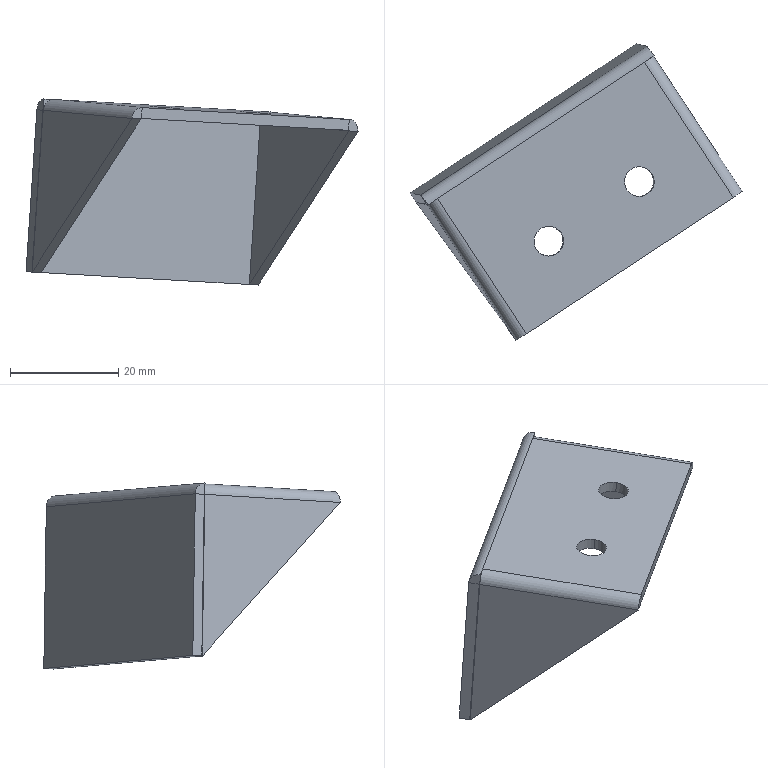Component | SolidWorks | LinearGuideRodSheetMetal-1 | 1 solid | 34 faces | box 61.25 x 54.67 x 34.32 mm | volume 7801 mm3 | plane 24 | cylinder 10 | commonest cylinder face diameters 5.5 x4 0.2 x3 4.2 x3 | material AISI 304
STEP:
#1=COLOUR_RGB('',0.7922,0.8196,0.9333);
#2=FILL_AREA_STYLE_COLOUR('',#1);
#3=FILL_AREA_STYLE('',(#2));
#4=SURFACE_STYLE_FILL_AREA(#3);
#5=SURFACE_SIDE_STYLE('',(#4));
#6=SURFACE_STYLE_USAGE(.BOTH.,#5);
#7=PRESENTATION_STYLE_ASSIGNMENT((#6));
#8=CARTESIAN_POINT('',(-6.363,-0.1525,32.19));
#9=VERTEX_POINT('',#8);
#10=CARTESIAN_POINT('',(-6.182,-0.03352,32.18));
#11=VERTEX_POINT('',#10);
#12=CARTESIAN_POINT('',(-6.272,-0.09302,32.185));
#13=DIRECTION('',(-0.0675,0.01553,-0.9976));
#14=DIRECTION('',(-0.8341,-0.5496,0.04788));
#15=AXIS2_PLACEMENT_3D('',#12,#13,#14);
#16=CIRCLE('',#15,0.1083);
#17=EDGE_CURVE('',#9,#11,#16,.T.);
#18=ORIENTED_EDGE('',*,*,#17,.T.);
#19=CARTESIAN_POINT('',(-6.177,-0.03474,32.258));
#20=VERTEX_POINT('',#19);
#21=CARTESIAN_POINT('',(-6.182,-0.03352,32.18));
#22=DIRECTION('',(0.0675,-0.01553,0.9976));
#23=VECTOR('',#22,39.37);
#24=LINE('',#21,#23);
#25=EDGE_CURVE('',#11,#20,#24,.T.);
#26=ORIENTED_EDGE('',*,*,#25,.T.);
#27=CARTESIAN_POINT('',(-6.357,-0.1537,32.269));
#28=VERTEX_POINT('',#27);
#29=CARTESIAN_POINT('',(-6.267,-0.09424,32.264));
#30=DIRECTION('',(-0.0675,0.01553,-0.9976));
#31=DIRECTION('',(-0.8341,-0.5496,0.04788));
#32=AXIS2_PLACEMENT_3D('',#29,#30,#31);
#33=CIRCLE('',#32,0.1083);
#34=EDGE_CURVE('',#28,#20,#33,.T.);
#35=ORIENTED_EDGE('',*,*,#34,.F.);
#36=CARTESIAN_POINT('',(-6.363,-0.1525,32.19));
#37=DIRECTION('',(0.0675,-0.01553,0.9976));
#38=VECTOR('',#37,39.37);
#39=LINE('',#36,#38);
#40=EDGE_CURVE('',#9,#28,#39,.T.);
#41=ORIENTED_EDGE('',*,*,#40,.F.);
#42=EDGE_LOOP('',(#18,#26,#35,#41));
#43=FACE_OUTER_BOUND('',#42,.T.);
#44=CARTESIAN_POINT('',(-6.272,-0.09302,32.185));
#45=DIRECTION('',(0.0675,-0.01553,0.9976));
#46=DIRECTION('',(-0.8341,-0.5496,0.04788));
#47=AXIS2_PLACEMENT_3D('',#44,#45,#46);
#48=CYLINDRICAL_SURFACE('',#47,0.1083);
#49=ADVANCED_FACE('',(#43),#48,.F.);
#50=CARTESIAN_POINT('',(-5.706,0.2802,32.152));
#51=VERTEX_POINT('',#50);
#52=CARTESIAN_POINT('',(-5.525,0.3992,32.142));
#53=VERTEX_POINT('',#52);
#54=CARTESIAN_POINT('',(-5.616,0.3397,32.147));
#55=DIRECTION('',(-0.0675,0.01553,-0.9976));
#56=DIRECTION('',(-0.8341,-0.5496,0.04788));
#57=AXIS2_PLACEMENT_3D('',#54,#55,#56);
#58=CIRCLE('',#57,0.1083);
#59=EDGE_CURVE('',#51,#53,#58,.T.);
#60=ORIENTED_EDGE('',*,*,#59,.T.);
#61=CARTESIAN_POINT('',(-5.52,0.398,32.221));
#62=VERTEX_POINT('',#61);
#63=CARTESIAN_POINT('',(-5.525,0.3992,32.142));
#64=DIRECTION('',(0.0675,-0.01553,0.9976));
#65=VECTOR('',#64,39.37);
#66=LINE('',#63,#65);
#67=EDGE_CURVE('',#53,#62,#66,.T.);
#68=ORIENTED_EDGE('',*,*,#67,.T.);
#69=CARTESIAN_POINT('',(-5.701,0.279,32.231));
#70=VERTEX_POINT('',#69);
#71=CARTESIAN_POINT('',(-5.61,0.3385,32.226));
#72=DIRECTION('',(-0.0675,0.01553,-0.9976));
#73=DIRECTION('',(-0.8341,-0.5496,0.04788));
#74=AXIS2_PLACEMENT_3D('',#71,#72,#73);
#75=CIRCLE('',#74,0.1083);
#76=EDGE_CURVE('',#70,#62,#75,.T.);
#77=ORIENTED_EDGE('',*,*,#76,.F.);
#78=CARTESIAN_POINT('',(-5.706,0.2802,32.152));
#79=DIRECTION('',(0.0675,-0.01553,0.9976));
#80=VECTOR('',#79,39.37);
#81=LINE('',#78,#80);
#82=EDGE_CURVE('',#51,#70,#81,.T.);
#83=ORIENTED_EDGE('',*,*,#82,.F.);
#84=EDGE_LOOP('',(#60,#68,#77,#83));
#85=FACE_OUTER_BOUND('',#84,.T.);
#86=CARTESIAN_POINT('',(-5.616,0.3397,32.147));
#87=DIRECTION('',(0.0675,-0.01553,0.9976));
#88=DIRECTION('',(-0.8341,-0.5496,0.04788));
#89=AXIS2_PLACEMENT_3D('',#86,#87,#88);
#90=CYLINDRICAL_SURFACE('',#89,0.1083);
#91=ADVANCED_FACE('',(#85),#90,.F.);
#92=CARTESIAN_POINT('',(-5.572,1.206,32.237));
#93=VERTEX_POINT('',#92);
#94=CARTESIAN_POINT('',(-5.504,1.252,32.233));
#95=VERTEX_POINT('',#94);
#96=CARTESIAN_POINT('',(-7.145,0.1699,32.327));
#97=DIRECTION('',(0.8341,0.5496,-0.04788));
#98=VECTOR('',#97,39.37);
#99=LINE('',#96,#98);
#100=EDGE_CURVE('',#93,#95,#99,.T.);
#101=ORIENTED_EDGE('',*,*,#100,.F.);
#102=CARTESIAN_POINT('',(-5.509,1.253,32.154));
#103=VERTEX_POINT('',#102);
#104=CARTESIAN_POINT('',(-5.578,1.208,32.154));
#105=DIRECTION('',(-0.5475,0.8353,0.05005));
#106=DIRECTION('',(0.8341,0.5496,-0.04788));
#107=AXIS2_PLACEMENT_3D('',#104,#105,#106);
#108=CIRCLE('',#107,0.08268);
#109=EDGE_CURVE('',#93,#103,#108,.T.);
#110=ORIENTED_EDGE('',*,*,#109,.T.);
#111=CARTESIAN_POINT('',(-5.509,1.253,32.154));
#112=VERTEX_POINT('',#111);
#113=CARTESIAN_POINT('',(-5.578,1.207,32.158));
#114=DIRECTION('',(0.8341,0.5496,-0.04788));
#115=VECTOR('',#114,39.37);
#116=LINE('',#113,#115);
#117=EDGE_CURVE('',#103,#112,#116,.T.);
#118=ORIENTED_EDGE('',*,*,#117,.T.);
#119=CARTESIAN_POINT('',(-5.509,1.253,32.154));
#120=DIRECTION('',(-0.0675,0.01553,-0.9976));
#121=VECTOR('',#120,39.37);
#122=LINE('',#119,#121);
#123=EDGE_CURVE('',#95,#112,#122,.T.);
#124=ORIENTED_EDGE('',*,*,#123,.F.);
#125=EDGE_LOOP('',(#101,#110,#118,#124));
#126=FACE_OUTER_BOUND('',#125,.T.);
#127=CARTESIAN_POINT('',(-5.578,1.207,32.158));
#128=DIRECTION('',(0.5475,-0.8353,-0.05005));
#129=DIRECTION('',(0.8341,0.5496,-0.04788));
#130=AXIS2_PLACEMENT_3D('',#127,#128,#129);
#131=PLANE('',#130);
#132=ADVANCED_FACE('',(#126),#131,.T.);
#133=CARTESIAN_POINT('',(-7.151,0.1711,32.249));
#134=VERTEX_POINT('',#133);
#135=CARTESIAN_POINT('',(-7.151,0.1711,32.249));
#136=VERTEX_POINT('',#135);
#137=CARTESIAN_POINT('',(-5.509,1.253,32.154));
#138=DIRECTION('',(0.8341,0.5496,-0.04788));
#139=VECTOR('',#138,39.37);
#140=LINE('',#137,#139);
#141=EDGE_CURVE('',#134,#136,#140,.T.);
#142=ORIENTED_EDGE('',*,*,#141,.T.);
#143=CARTESIAN_POINT('',(-7.076,0.2153,32.323));
#144=VERTEX_POINT('',#143);
#145=CARTESIAN_POINT('',(-7.082,0.2166,32.241));
#146=DIRECTION('',(-0.5475,0.8353,0.05005));
#147=DIRECTION('',(-0.8341,-0.5496,0.04788));
#148=AXIS2_PLACEMENT_3D('',#145,#146,#147);
#149=CIRCLE('',#148,0.08268);
#150=EDGE_CURVE('',#136,#144,#149,.T.);
#151=ORIENTED_EDGE('',*,*,#150,.T.);
#152=CARTESIAN_POINT('',(-7.145,0.1699,32.327));
#153=VERTEX_POINT('',#152);
#154=CARTESIAN_POINT('',(-7.145,0.1699,32.327));
#155=DIRECTION('',(0.8341,0.5496,-0.04788));
#156=VECTOR('',#155,39.37);
#157=LINE('',#154,#156);
#158=EDGE_CURVE('',#153,#144,#157,.T.);
#159=ORIENTED_EDGE('',*,*,#158,.F.);
#160=CARTESIAN_POINT('',(-7.151,0.1711,32.249));
#161=DIRECTION('',(-0.0675,0.01553,-0.9976));
#162=VECTOR('',#161,39.37);
#163=LINE('',#160,#162);
#164=EDGE_CURVE('',#153,#134,#163,.T.);
#165=ORIENTED_EDGE('',*,*,#164,.T.);
#166=EDGE_LOOP('',(#142,#151,#159,#165));
#167=FACE_OUTER_BOUND('',#166,.T.);
#168=CARTESIAN_POINT('',(-7.151,0.1711,32.249));
#169=DIRECTION('',(0.5475,-0.8353,-0.05005));
#170=DIRECTION('',(0.8341,0.5496,-0.04788));
#171=AXIS2_PLACEMENT_3D('',#168,#169,#170);
#172=PLANE('',#171);
#173=ADVANCED_FACE('',(#167),#172,.T.);
#174=ORIENTED_EDGE('',*,*,#59,.F.);
#175=CARTESIAN_POINT('',(-5.616,0.3397,32.147));
#176=DIRECTION('',(-0.0675,0.01553,-0.9976));
#177=DIRECTION('',(-0.8341,-0.5496,0.04788));
#178=AXIS2_PLACEMENT_3D('',#175,#176,#177);
#179=CIRCLE('',#178,0.1083);
#180=EDGE_CURVE('',#53,#51,#179,.T.);
#181=ORIENTED_EDGE('',*,*,#180,.F.);
#182=EDGE_LOOP('',(#174,#181));
#183=FACE_BOUND('',#182,.T.);
#184=ORIENTED_EDGE('',*,*,#17,.F.);
#185=CARTESIAN_POINT('',(-6.272,-0.09302,32.185));
#186=DIRECTION('',(-0.0675,0.01553,-0.9976));
#187=DIRECTION('',(-0.8341,-0.5496,0.04788));
#188=AXIS2_PLACEMENT_3D('',#185,#186,#187);
#189=CIRCLE('',#188,0.1083);
#190=EDGE_CURVE('',#11,#9,#189,.T.);
#191=ORIENTED_EDGE('',*,*,#190,.F.);
#192=EDGE_LOOP('',(#184,#191));
#193=FACE_BOUND('',#192,.T.);
#194=CARTESIAN_POINT('',(-4.933,0.2242,32.099));
#195=VERTEX_POINT('',#194);
#196=CARTESIAN_POINT('',(-5.578,1.207,32.158));
#197=VERTEX_POINT('',#196);
#198=CARTESIAN_POINT('',(-4.933,0.2242,32.099));
#199=DIRECTION('',(-0.5475,0.8353,0.05005));
#200=VECTOR('',#199,39.37);
#201=LINE('',#198,#200);
#202=EDGE_CURVE('',#195,#197,#201,.T.);
#203=ORIENTED_EDGE('',*,*,#202,.F.);
#204=CARTESIAN_POINT('',(-6.437,-0.7668,32.186));
#205=VERTEX_POINT('',#204);
#206=CARTESIAN_POINT('',(-6.506,-0.8122,32.19));
#207=DIRECTION('',(0.8341,0.5496,-0.04788));
#208=VECTOR('',#207,39.37);
#209=LINE('',#206,#208);
#210=EDGE_CURVE('',#205,#195,#209,.T.);
#211=ORIENTED_EDGE('',*,*,#210,.F.);
#212=CARTESIAN_POINT('',(-7.082,0.2165,32.245));
#213=VERTEX_POINT('',#212);
#214=CARTESIAN_POINT('',(-7.082,0.2165,32.245));
#215=DIRECTION('',(0.5475,-0.8353,-0.05005));
#216=VECTOR('',#215,39.37);
#217=LINE('',#214,#216);
#218=EDGE_CURVE('',#213,#205,#217,.T.);
#219=ORIENTED_EDGE('',*,*,#218,.F.);
#220=CARTESIAN_POINT('',(-5.509,1.253,32.154));
#221=DIRECTION('',(0.8341,0.5496,-0.04788));
#222=VECTOR('',#221,39.37);
#223=LINE('',#220,#222);
#224=EDGE_CURVE('',#213,#197,#223,.T.);
#225=ORIENTED_EDGE('',*,*,#224,.T.);
#226=EDGE_LOOP('',(#203,#211,#219,#225));
#227=FACE_OUTER_BOUND('',#226,.T.);
#228=CARTESIAN_POINT('',(-7.153,0.1744,32.249));
#229=DIRECTION('',(0.0675,-0.01553,0.9976));
#230=DIRECTION('',(-0.8341,-0.5496,0.04788));
#231=AXIS2_PLACEMENT_3D('',#228,#229,#230);
#232=PLANE('',#231);
#233=ADVANCED_FACE('',(#183,#193,#227),#232,.F.);
#234=ORIENTED_EDGE('',*,*,#76,.T.);
#235=CARTESIAN_POINT('',(-5.61,0.3385,32.226));
#236=DIRECTION('',(-0.0675,0.01553,-0.9976));
#237=DIRECTION('',(-0.8341,-0.5496,0.04788));
#238=AXIS2_PLACEMENT_3D('',#235,#236,#237);
#239=CIRCLE('',#238,0.1083);
#240=EDGE_CURVE('',#62,#70,#239,.T.);
#241=ORIENTED_EDGE('',*,*,#240,.T.);
#242=EDGE_LOOP('',(#234,#241));
#243=FACE_BOUND('',#242,.T.);
#244=ORIENTED_EDGE('',*,*,#34,.T.);
#245=CARTESIAN_POINT('',(-6.267,-0.09424,32.264));
#246=DIRECTION('',(-0.0675,0.01553,-0.9976));
#247=DIRECTION('',(-0.8341,-0.5496,0.04788));
#248=AXIS2_PLACEMENT_3D('',#245,#246,#247);
#249=CIRCLE('',#248,0.1083);
#250=EDGE_CURVE('',#20,#28,#249,.T.);
#251=ORIENTED_EDGE('',*,*,#250,.T.);
#252=EDGE_LOOP('',(#244,#251));
#253=FACE_BOUND('',#252,.T.);
#254=CARTESIAN_POINT('',(-6.432,-0.768,32.264));
#255=VERTEX_POINT('',#254);
#256=CARTESIAN_POINT('',(-4.928,0.223,32.178));
#257=VERTEX_POINT('',#256);
#258=CARTESIAN_POINT('',(-6.501,-0.8134,32.268));
#259=DIRECTION('',(0.8341,0.5496,-0.04788));
#260=VECTOR('',#259,39.37);
#261=LINE('',#258,#260);
#262=EDGE_CURVE('',#255,#257,#261,.T.);
#263=ORIENTED_EDGE('',*,*,#262,.T.);
#264=CARTESIAN_POINT('',(-4.928,0.223,32.178));
#265=DIRECTION('',(-0.5475,0.8353,0.05005));
#266=VECTOR('',#265,39.37);
#267=LINE('',#264,#266);
#268=EDGE_CURVE('',#257,#93,#267,.T.);
#269=ORIENTED_EDGE('',*,*,#268,.T.);
#270=CARTESIAN_POINT('',(-7.145,0.1699,32.327));
#271=DIRECTION('',(0.8341,0.5496,-0.04788));
#272=VECTOR('',#271,39.37);
#273=LINE('',#270,#272);
#274=EDGE_CURVE('',#144,#93,#273,.T.);
#275=ORIENTED_EDGE('',*,*,#274,.F.);
#276=CARTESIAN_POINT('',(-7.076,0.2153,32.323));
#277=DIRECTION('',(0.5475,-0.8353,-0.05005));
#278=VECTOR('',#277,39.37);
#279=LINE('',#276,#278);
#280=EDGE_CURVE('',#144,#255,#279,.T.);
#281=ORIENTED_EDGE('',*,*,#280,.T.);
#282=EDGE_LOOP('',(#263,#269,#275,#281));
#283=FACE_OUTER_BOUND('',#282,.T.);
#284=CARTESIAN_POINT('',(-7.148,0.1731,32.327));
#285=DIRECTION('',(0.0675,-0.01553,0.9976));
#286=DIRECTION('',(-0.8341,-0.5496,0.04788));
#287=AXIS2_PLACEMENT_3D('',#284,#285,#286);
#288=PLANE('',#287);
#289=ADVANCED_FACE('',(#243,#253,#283),#288,.T.);
#290=ORIENTED_EDGE('',*,*,#210,.T.);
#291=CARTESIAN_POINT('',(-4.933,0.2242,32.099));
#292=DIRECTION('',(0.0675,-0.01553,0.9976));
#293=VECTOR('',#292,39.37);
#294=LINE('',#291,#293);
#295=EDGE_CURVE('',#195,#257,#294,.T.);
#296=ORIENTED_EDGE('',*,*,#295,.T.);
#297=ORIENTED_EDGE('',*,*,#262,.F.);
#298=CARTESIAN_POINT('',(-6.437,-0.7668,32.186));
#299=DIRECTION('',(0.0675,-0.01553,0.9976));
#300=VECTOR('',#299,39.37);
#301=LINE('',#298,#300);
#302=EDGE_CURVE('',#205,#255,#301,.T.);
#303=ORIENTED_EDGE('',*,*,#302,.F.);
#304=EDGE_LOOP('',(#290,#296,#297,#303));
#305=FACE_OUTER_BOUND('',#304,.T.);
#306=CARTESIAN_POINT('',(-6.506,-0.8122,32.19));
#307=DIRECTION('',(0.5475,-0.8353,-0.05005));
#308=DIRECTION('',(0.8341,0.5496,-0.04788));
#309=AXIS2_PLACEMENT_3D('',#306,#307,#308);
#310=PLANE('',#309);
#311=ADVANCED_FACE('',(#305),#310,.T.);
#312=ORIENTED_EDGE('',*,*,#164,.F.);
#313=CARTESIAN_POINT('',(-7.196,0.2402,32.249));
#314=VERTEX_POINT('',#313);
#315=CARTESIAN_POINT('',(-7.151,0.1711,32.245));
#316=DIRECTION('',(-0.8341,-0.5496,0.04788));
#317=DIRECTION('',(0.5475,-0.8353,-0.05005));
#318=AXIS2_PLACEMENT_3D('',#315,#316,#317);
#319=CIRCLE('',#318,0.08268);
#320=EDGE_CURVE('',#153,#314,#319,.T.);
#321=ORIENTED_EDGE('',*,*,#320,.T.);
#322=CARTESIAN_POINT('',(-7.153,0.1744,32.245));
#323=VERTEX_POINT('',#322);
#324=CARTESIAN_POINT('',(-7.153,0.1744,32.245));
#325=DIRECTION('',(0.5475,-0.8353,-0.05005));
#326=VECTOR('',#325,39.37);
#327=LINE('',#324,#326);
#328=EDGE_CURVE('',#314,#323,#327,.T.);
#329=ORIENTED_EDGE('',*,*,#328,.T.);
#330=CARTESIAN_POINT('',(-7.151,0.1711,32.245));
#331=DIRECTION('',(-0.8341,-0.5496,0.04788));
#332=DIRECTION('',(-0.5475,0.8353,0.05005));
#333=AXIS2_PLACEMENT_3D('',#330,#331,#332);
#334=CIRCLE('',#333,0.003937);
#335=EDGE_CURVE('',#134,#323,#334,.T.);
#336=ORIENTED_EDGE('',*,*,#335,.F.);
#337=EDGE_LOOP('',(#312,#321,#329,#336));
#338=FACE_OUTER_BOUND('',#337,.T.);
#339=CARTESIAN_POINT('',(-7.151,0.1711,32.245));
#340=DIRECTION('',(-0.8341,-0.5496,0.04788));
#341=DIRECTION('',(0.5475,-0.8353,-0.05005));
#342=AXIS2_PLACEMENT_3D('',#339,#340,#341);
#343=PLANE('',#342);
#344=ADVANCED_FACE('',(#338),#343,.T.);
#345=ORIENTED_EDGE('',*,*,#328,.F.);
#346=CARTESIAN_POINT('',(-7.276,0.2585,31.074));
#347=VERTEX_POINT('',#346);
#348=CARTESIAN_POINT('',(-7.196,0.2401,32.253));
#349=DIRECTION('',(0.0675,-0.01553,0.9976));
#350=VECTOR('',#349,39.37);
#351=LINE('',#348,#350);
#352=EDGE_CURVE('',#347,#314,#351,.T.);
#353=ORIENTED_EDGE('',*,*,#352,.F.);
#354=CARTESIAN_POINT('',(-7.233,0.1927,31.07));
#355=VERTEX_POINT('',#354);
#356=CARTESIAN_POINT('',(-7.233,0.1927,31.07));
#357=DIRECTION('',(0.5475,-0.8353,-0.05005));
#358=VECTOR('',#357,39.37);
#359=LINE('',#356,#358);
#360=EDGE_CURVE('',#347,#355,#359,.T.);
#361=ORIENTED_EDGE('',*,*,#360,.T.);
#362=CARTESIAN_POINT('',(-7.153,0.1744,32.249));
#363=DIRECTION('',(0.0675,-0.01553,0.9976));
#364=VECTOR('',#363,39.37);
#365=LINE('',#362,#364);
#366=EDGE_CURVE('',#355,#323,#365,.T.);
#367=ORIENTED_EDGE('',*,*,#366,.T.);
#368=EDGE_LOOP('',(#345,#353,#361,#367));
#369=FACE_OUTER_BOUND('',#368,.T.);
#370=CARTESIAN_POINT('',(-7.153,0.1744,32.249));
#371=DIRECTION('',(-0.8341,-0.5496,0.04788));
#372=DIRECTION('',(0.0675,-0.01553,0.9976));
#373=AXIS2_PLACEMENT_3D('',#370,#371,#372);
#374=PLANE('',#373);
#375=ADVANCED_FACE('',(#369),#374,.T.);
#376=ORIENTED_EDGE('',*,*,#360,.F.);
#377=CARTESIAN_POINT('',(-5.634,1.34,30.98));
#378=VERTEX_POINT('',#377);
#379=CARTESIAN_POINT('',(-7.276,0.2585,31.074));
#380=DIRECTION('',(0.8341,0.5496,-0.04788));
#381=VECTOR('',#380,39.37);
#382=LINE('',#379,#381);
#383=EDGE_CURVE('',#347,#378,#382,.T.);
#384=ORIENTED_EDGE('',*,*,#383,.T.);
#385=CARTESIAN_POINT('',(-5.591,1.275,30.976));
#386=VERTEX_POINT('',#385);
#387=CARTESIAN_POINT('',(-5.591,1.275,30.976));
#388=DIRECTION('',(0.5475,-0.8353,-0.05005));
#389=VECTOR('',#388,39.37);
#390=LINE('',#387,#389);
#391=EDGE_CURVE('',#378,#386,#390,.T.);
#392=ORIENTED_EDGE('',*,*,#391,.T.);
#393=CARTESIAN_POINT('',(-7.233,0.1927,31.07));
#394=DIRECTION('',(0.8341,0.5496,-0.04788));
#395=VECTOR('',#394,39.37);
#396=LINE('',#393,#395);
#397=EDGE_CURVE('',#355,#386,#396,.T.);
#398=ORIENTED_EDGE('',*,*,#397,.F.);
#399=EDGE_LOOP('',(#376,#384,#392,#398));
#400=FACE_OUTER_BOUND('',#399,.T.);
#401=CARTESIAN_POINT('',(-7.233,0.1927,31.07));
#402=DIRECTION('',(0.0675,-0.01553,0.9976));
#403=DIRECTION('',(0.8341,0.5496,-0.04788));
#404=AXIS2_PLACEMENT_3D('',#401,#402,#403);
#405=PLANE('',#404);
#406=ADVANCED_FACE('',(#400),#405,.F.);
#407=ORIENTED_EDGE('',*,*,#391,.F.);
#408=CARTESIAN_POINT('',(-5.554,1.322,32.154));
#409=VERTEX_POINT('',#408);
#410=CARTESIAN_POINT('',(-5.554,1.322,32.158));
#411=DIRECTION('',(0.0675,-0.01553,0.9976));
#412=VECTOR('',#411,39.37);
#413=LINE('',#410,#412);
#414=EDGE_CURVE('',#378,#409,#413,.T.);
#415=ORIENTED_EDGE('',*,*,#414,.T.);
#416=CARTESIAN_POINT('',(-5.511,1.256,32.151));
#417=VERTEX_POINT('',#416);
#418=CARTESIAN_POINT('',(-5.511,1.256,32.151));
#419=DIRECTION('',(0.5475,-0.8353,-0.05005));
#420=VECTOR('',#419,39.37);
#421=LINE('',#418,#420);
#422=EDGE_CURVE('',#409,#417,#421,.T.);
#423=ORIENTED_EDGE('',*,*,#422,.T.);
#424=CARTESIAN_POINT('',(-5.511,1.256,32.154));
#425=DIRECTION('',(0.0675,-0.01553,0.9976));
#426=VECTOR('',#425,39.37);
#427=LINE('',#424,#426);
#428=EDGE_CURVE('',#386,#417,#427,.T.);
#429=ORIENTED_EDGE('',*,*,#428,.F.);
#430=EDGE_LOOP('',(#407,#415,#423,#429));
#431=FACE_OUTER_BOUND('',#430,.T.);
#432=CARTESIAN_POINT('',(-5.511,1.256,32.154));
#433=DIRECTION('',(-0.8341,-0.5496,0.04788));
#434=DIRECTION('',(0.0675,-0.01553,0.9976));
#435=AXIS2_PLACEMENT_3D('',#432,#433,#434);
#436=PLANE('',#435);
#437=ADVANCED_FACE('',(#431),#436,.F.);
#438=ORIENTED_EDGE('',*,*,#67,.F.);
#439=ORIENTED_EDGE('',*,*,#180,.T.);
#440=ORIENTED_EDGE('',*,*,#82,.T.);
#441=ORIENTED_EDGE('',*,*,#240,.F.);
#442=EDGE_LOOP('',(#438,#439,#440,#441));
#443=FACE_OUTER_BOUND('',#442,.T.);
#444=CARTESIAN_POINT('',(-5.616,0.3397,32.147));
#445=DIRECTION('',(0.0675,-0.01553,0.9976));
#446=DIRECTION('',(-0.8341,-0.5496,0.04788));
#447=AXIS2_PLACEMENT_3D('',#444,#445,#446);
#448=CYLINDRICAL_SURFACE('',#447,0.1083);
#449=ADVANCED_FACE('',(#443),#448,.F.);
#450=ORIENTED_EDGE('',*,*,#25,.F.);
#451=ORIENTED_EDGE('',*,*,#190,.T.);
#452=ORIENTED_EDGE('',*,*,#40,.T.);
#453=ORIENTED_EDGE('',*,*,#250,.F.);
#454=EDGE_LOOP('',(#450,#451,#452,#453));
#455=FACE_OUTER_BOUND('',#454,.T.);
#456=CARTESIAN_POINT('',(-6.272,-0.09302,32.185));
#457=DIRECTION('',(0.0675,-0.01553,0.9976));
#458=DIRECTION('',(-0.8341,-0.5496,0.04788));
#459=AXIS2_PLACEMENT_3D('',#456,#457,#458);
#460=CYLINDRICAL_SURFACE('',#459,0.1083);
#461=ADVANCED_FACE('',(#455),#460,.F.);
#462=CARTESIAN_POINT('',(-5.509,1.253,32.15));
#463=DIRECTION('',(0.8341,0.5496,-0.04788));
#464=DIRECTION('',(0.5475,-0.8353,-0.05005));
#465=AXIS2_PLACEMENT_3D('',#462,#463,#464);
#466=CIRCLE('',#465,0.08268);
#467=EDGE_CURVE('',#409,#95,#466,.T.);
#468=ORIENTED_EDGE('',*,*,#467,.T.);
#469=ORIENTED_EDGE('',*,*,#123,.T.);
#470=CARTESIAN_POINT('',(-5.509,1.253,32.15));
#471=DIRECTION('',(0.8341,0.5496,-0.04788));
#472=DIRECTION('',(0.5475,-0.8353,-0.05005));
#473=AXIS2_PLACEMENT_3D('',#470,#471,#472);
#474=CIRCLE('',#473,0.003937);
#475=EDGE_CURVE('',#417,#112,#474,.T.);
#476=ORIENTED_EDGE('',*,*,#475,.F.);
#477=ORIENTED_EDGE('',*,*,#422,.F.);
#478=EDGE_LOOP('',(#468,#469,#476,#477));
#479=FACE_OUTER_BOUND('',#478,.T.);
#480=CARTESIAN_POINT('',(-5.509,1.253,32.15));
#481=DIRECTION('',(0.8341,0.5496,-0.04788));
#482=DIRECTION('',(-0.5475,0.8353,0.05005));
#483=AXIS2_PLACEMENT_3D('',#480,#481,#482);
#484=PLANE('',#483);
#485=ADVANCED_FACE('',(#479),#484,.T.);
#486=ORIENTED_EDGE('',*,*,#428,.T.);
#487=CARTESIAN_POINT('',(-7.153,0.1744,32.245));
#488=DIRECTION('',(-0.8341,-0.5496,0.04788));
#489=VECTOR('',#488,39.37);
#490=LINE('',#487,#489);
#491=EDGE_CURVE('',#417,#323,#490,.T.);
#492=ORIENTED_EDGE('',*,*,#491,.T.);
#493=ORIENTED_EDGE('',*,*,#366,.F.);
#494=ORIENTED_EDGE('',*,*,#397,.T.);
#495=EDGE_LOOP('',(#486,#492,#493,#494));
#496=FACE_OUTER_BOUND('',#495,.T.);
#497=CARTESIAN_POINT('',(-7.153,0.1744,32.249));
#498=DIRECTION('',(-0.5475,0.8353,0.05005));
#499=DIRECTION('',(-0.0675,0.01553,-0.9976));
#500=AXIS2_PLACEMENT_3D('',#497,#498,#499);
#501=PLANE('',#500);
#502=ADVANCED_FACE('',(#496),#501,.F.);
#503=ORIENTED_EDGE('',*,*,#335,.T.);
#504=ORIENTED_EDGE('',*,*,#491,.F.);
#505=ORIENTED_EDGE('',*,*,#475,.T.);
#506=ORIENTED_EDGE('',*,*,#117,.F.);
#507=CARTESIAN_POINT('',(-5.578,1.207,32.158));
#508=DIRECTION('',(0.8341,0.5496,-0.04788));
#509=VECTOR('',#508,39.37);
#510=LINE('',#507,#509);
#511=EDGE_CURVE('',#197,#103,#510,.T.);
#512=ORIENTED_EDGE('',*,*,#511,.F.);
#513=ORIENTED_EDGE('',*,*,#224,.F.);
#514=CARTESIAN_POINT('',(-5.509,1.253,32.154));
#515=DIRECTION('',(0.8341,0.5496,-0.04788));
#516=VECTOR('',#515,39.37);
#517=LINE('',#514,#516);
#518=EDGE_CURVE('',#136,#213,#517,.T.);
#519=ORIENTED_EDGE('',*,*,#518,.F.);
#520=ORIENTED_EDGE('',*,*,#141,.F.);
#521=EDGE_LOOP('',(#503,#504,#505,#506,#512,#513,#519,#520));
#522=FACE_OUTER_BOUND('',#521,.T.);
#523=CARTESIAN_POINT('',(-7.151,0.1711,32.245));
#524=DIRECTION('',(-0.8341,-0.5496,0.04788));
#525=DIRECTION('',(0.5475,-0.8353,-0.05005));
#526=AXIS2_PLACEMENT_3D('',#523,#524,#525);
#527=CYLINDRICAL_SURFACE('',#526,0.003937);
#528=ADVANCED_FACE('',(#522),#527,.F.);
#529=ORIENTED_EDGE('',*,*,#414,.F.);
#530=ORIENTED_EDGE('',*,*,#383,.F.);
#531=ORIENTED_EDGE('',*,*,#352,.T.);
#532=CARTESIAN_POINT('',(-7.196,0.2402,32.249));
#533=DIRECTION('',(-0.8341,-0.5496,0.04788));
#534=VECTOR('',#533,39.37);
#535=LINE('',#532,#534);
#536=EDGE_CURVE('',#409,#314,#535,.T.);
#537=ORIENTED_EDGE('',*,*,#536,.F.);
#538=EDGE_LOOP('',(#529,#530,#531,#537));
#539=FACE_OUTER_BOUND('',#538,.T.);
#540=CARTESIAN_POINT('',(-7.196,0.2401,32.253));
#541=DIRECTION('',(-0.5475,0.8353,0.05005));
#542=DIRECTION('',(-0.0675,0.01553,-0.9976));
#543=AXIS2_PLACEMENT_3D('',#540,#541,#542);
#544=PLANE('',#543);
#545=ADVANCED_FACE('',(#539),#544,.T.);
#546=ORIENTED_EDGE('',*,*,#320,.F.);
#547=ORIENTED_EDGE('',*,*,#158,.T.);
#548=ORIENTED_EDGE('',*,*,#274,.T.);
#549=ORIENTED_EDGE('',*,*,#100,.T.);
#550=ORIENTED_EDGE('',*,*,#467,.F.);
#551=ORIENTED_EDGE('',*,*,#536,.T.);
#552=EDGE_LOOP('',(#546,#547,#548,#549,#550,#551));
#553=FACE_OUTER_BOUND('',#552,.T.);
#554=CARTESIAN_POINT('',(-7.151,0.1711,32.245));
#555=DIRECTION('',(-0.8341,-0.5496,0.04788));
#556=DIRECTION('',(0.5475,-0.8353,-0.05005));
#557=AXIS2_PLACEMENT_3D('',#554,#555,#556);
#558=CYLINDRICAL_SURFACE('',#557,0.08268);
#559=ADVANCED_FACE('',(#553),#558,.T.);
#560=CARTESIAN_POINT('',(-6.441,-0.7689,32.182));
#561=VERTEX_POINT('',#560);
#562=CARTESIAN_POINT('',(-6.506,-0.8121,32.186));
#563=VERTEX_POINT('',#562);
#564=CARTESIAN_POINT('',(-6.506,-0.8121,32.186));
#565=DIRECTION('',(-0.8341,-0.5496,0.04788));
#566=VECTOR('',#565,39.37);
#567=LINE('',#564,#566);
#568=EDGE_CURVE('',#561,#563,#567,.T.);
#569=ORIENTED_EDGE('',*,*,#568,.F.);
#570=CARTESIAN_POINT('',(-6.437,-0.7667,32.182));
#571=DIRECTION('',(0.5475,-0.8353,-0.05005));
#572=DIRECTION('',(-0.8341,-0.5496,0.04788));
#573=AXIS2_PLACEMENT_3D('',#570,#571,#572);
#574=CIRCLE('',#573,0.003937);
#575=EDGE_CURVE('',#205,#561,#574,.T.);
#576=ORIENTED_EDGE('',*,*,#575,.F.);
#577=ORIENTED_EDGE('',*,*,#302,.T.);
#578=CARTESIAN_POINT('',(-6.437,-0.7667,32.182));
#579=DIRECTION('',(0.5475,-0.8353,-0.05005));
#580=DIRECTION('',(-0.8341,-0.5496,0.04788));
#581=AXIS2_PLACEMENT_3D('',#578,#579,#580);
#582=CIRCLE('',#581,0.08268);
#583=EDGE_CURVE('',#255,#563,#582,.T.);
#584=ORIENTED_EDGE('',*,*,#583,.T.);
#585=EDGE_LOOP('',(#569,#576,#577,#584));
#586=FACE_OUTER_BOUND('',#585,.T.);
#587=CARTESIAN_POINT('',(-6.437,-0.7667,32.182));
#588=DIRECTION('',(0.5475,-0.8353,-0.05005));
#589=DIRECTION('',(0.8341,0.5496,-0.04788));
#590=AXIS2_PLACEMENT_3D('',#587,#588,#589);
#591=PLANE('',#590);
#592=ADVANCED_FACE('',(#586),#591,.T.);
#593=CARTESIAN_POINT('',(-7.151,0.1711,32.245));
#594=VERTEX_POINT('',#593);
#595=CARTESIAN_POINT('',(-7.082,0.2166,32.241));
#596=DIRECTION('',(-0.5475,0.8353,0.05005));
#597=DIRECTION('',(-0.8341,-0.5496,0.04788));
#598=AXIS2_PLACEMENT_3D('',#595,#596,#597);
#599=CIRCLE('',#598,0.08268);
#600=EDGE_CURVE('',#594,#136,#599,.T.);
#601=ORIENTED_EDGE('',*,*,#600,.T.);
#602=ORIENTED_EDGE('',*,*,#518,.T.);
#603=CARTESIAN_POINT('',(-7.085,0.2144,32.241));
#604=VERTEX_POINT('',#603);
#605=CARTESIAN_POINT('',(-7.082,0.2166,32.241));
#606=DIRECTION('',(-0.5475,0.8353,0.05005));
#607=DIRECTION('',(-0.8341,-0.5496,0.04788));
#608=AXIS2_PLACEMENT_3D('',#605,#606,#607);
#609=CIRCLE('',#608,0.003937);
#610=EDGE_CURVE('',#604,#213,#609,.T.);
#611=ORIENTED_EDGE('',*,*,#610,.F.);
#612=CARTESIAN_POINT('',(-7.085,0.2144,32.241));
#613=DIRECTION('',(-0.8341,-0.5496,0.04788));
#614=VECTOR('',#613,39.37);
#615=LINE('',#612,#614);
#616=EDGE_CURVE('',#604,#594,#615,.T.);
#617=ORIENTED_EDGE('',*,*,#616,.T.);
#618=EDGE_LOOP('',(#601,#602,#611,#617));
#619=FACE_OUTER_BOUND('',#618,.T.);
#620=CARTESIAN_POINT('',(-7.082,0.2166,32.241));
#621=DIRECTION('',(0.5475,-0.8353,-0.05005));
#622=DIRECTION('',(0.8341,0.5496,-0.04788));
#623=AXIS2_PLACEMENT_3D('',#620,#621,#622);
#624=PLANE('',#623);
#625=ADVANCED_FACE('',(#619),#624,.F.);
#626=ORIENTED_EDGE('',*,*,#280,.F.);
#627=ORIENTED_EDGE('',*,*,#150,.F.);
#628=ORIENTED_EDGE('',*,*,#600,.F.);
#629=CARTESIAN_POINT('',(-7.153,0.1744,32.245));
#630=DIRECTION('',(-0.5475,0.8353,0.05005));
#631=VECTOR('',#630,39.37);
#632=LINE('',#629,#631);
#633=EDGE_CURVE('',#563,#594,#632,.T.);
#634=ORIENTED_EDGE('',*,*,#633,.F.);
#635=ORIENTED_EDGE('',*,*,#583,.F.);
#636=EDGE_LOOP('',(#626,#627,#628,#634,#635));
#637=FACE_OUTER_BOUND('',#636,.T.);
#638=CARTESIAN_POINT('',(-7.082,0.2166,32.241));
#639=DIRECTION('',(-0.5475,0.8353,0.05005));
#640=DIRECTION('',(-0.8341,-0.5496,0.04788));
#641=AXIS2_PLACEMENT_3D('',#638,#639,#640);
#642=CYLINDRICAL_SURFACE('',#641,0.08268);
#643=ADVANCED_FACE('',(#637),#642,.T.);
#644=ORIENTED_EDGE('',*,*,#218,.T.);
#645=ORIENTED_EDGE('',*,*,#575,.T.);
#646=CARTESIAN_POINT('',(-6.441,-0.7689,32.182));
#647=DIRECTION('',(-0.5475,0.8353,0.05005));
#648=VECTOR('',#647,39.37);
#649=LINE('',#646,#648);
#650=EDGE_CURVE('',#561,#604,#649,.T.);
#651=ORIENTED_EDGE('',*,*,#650,.T.);
#652=ORIENTED_EDGE('',*,*,#610,.T.);
#653=EDGE_LOOP('',(#644,#645,#651,#652));
#654=FACE_OUTER_BOUND('',#653,.T.);
#655=CARTESIAN_POINT('',(-7.082,0.2166,32.241));
#656=DIRECTION('',(-0.5475,0.8353,0.05005));
#657=DIRECTION('',(-0.8341,-0.5496,0.04788));
#658=AXIS2_PLACEMENT_3D('',#655,#656,#657);
#659=CYLINDRICAL_SURFACE('',#658,0.003937);
#660=ADVANCED_FACE('',(#654),#659,.F.);
#661=CARTESIAN_POINT('',(-7.23,0.1894,31.07));
#662=VERTEX_POINT('',#661);
#663=CARTESIAN_POINT('',(-7.151,0.1711,32.249));
#664=DIRECTION('',(0.0675,-0.01553,0.9976));
#665=VECTOR('',#664,39.37);
#666=LINE('',#663,#665);
#667=EDGE_CURVE('',#662,#594,#666,.T.);
#668=ORIENTED_EDGE('',*,*,#667,.T.);
#669=ORIENTED_EDGE('',*,*,#616,.F.);
#670=CARTESIAN_POINT('',(-7.165,0.2327,31.066));
#671=VERTEX_POINT('',#670);
#672=CARTESIAN_POINT('',(-7.085,0.2143,32.245));
#673=DIRECTION('',(0.0675,-0.01553,0.9976));
#674=VECTOR('',#673,39.37);
#675=LINE('',#672,#674);
#676=EDGE_CURVE('',#671,#604,#675,.T.);
#677=ORIENTED_EDGE('',*,*,#676,.F.);
#678=CARTESIAN_POINT('',(-7.23,0.1894,31.07));
#679=DIRECTION('',(0.8341,0.5496,-0.04788));
#680=VECTOR('',#679,39.37);
#681=LINE('',#678,#680);
#682=EDGE_CURVE('',#662,#671,#681,.T.);
#683=ORIENTED_EDGE('',*,*,#682,.F.);
#684=EDGE_LOOP('',(#668,#669,#677,#683));
#685=FACE_OUTER_BOUND('',#684,.T.);
#686=CARTESIAN_POINT('',(-7.151,0.1711,32.249));
#687=DIRECTION('',(-0.5475,0.8353,0.05005));
#688=DIRECTION('',(-0.8341,-0.5496,0.04788));
#689=AXIS2_PLACEMENT_3D('',#686,#687,#688);
#690=PLANE('',#689);
#691=ADVANCED_FACE('',(#685),#690,.T.);
#692=CARTESIAN_POINT('',(-6.506,-0.8121,32.186));
#693=DIRECTION('',(-0.4349,0.6016,-0.67));
#694=VECTOR('',#693,39.37);
#695=LINE('',#692,#694);
#696=EDGE_CURVE('',#563,#662,#695,.T.);
#697=ORIENTED_EDGE('',*,*,#696,.F.);
#698=ORIENTED_EDGE('',*,*,#633,.T.);
#699=ORIENTED_EDGE('',*,*,#667,.F.);
#700=EDGE_LOOP('',(#697,#698,#699));
#701=FACE_OUTER_BOUND('',#700,.T.);
#702=CARTESIAN_POINT('',(-7.153,0.1744,32.249));
#703=DIRECTION('',(-0.8341,-0.5496,0.04788));
#704=DIRECTION('',(-0.0675,0.01553,-0.9976));
#705=AXIS2_PLACEMENT_3D('',#702,#703,#704);
#706=PLANE('',#705);
#707=ADVANCED_FACE('',(#701),#706,.T.);
#708=ORIENTED_EDGE('',*,*,#650,.F.);
#709=CARTESIAN_POINT('',(-6.803,-0.2681,31.624));
#710=DIRECTION('',(-0.4349,0.6016,-0.67));
#711=VECTOR('',#710,39.37);
#712=LINE('',#709,#711);
#713=EDGE_CURVE('',#561,#671,#712,.T.);
#714=ORIENTED_EDGE('',*,*,#713,.T.);
#715=ORIENTED_EDGE('',*,*,#676,.T.);
#716=EDGE_LOOP('',(#708,#714,#715));
#717=FACE_OUTER_BOUND('',#716,.T.);
#718=CARTESIAN_POINT('',(-7.087,0.2176,32.245));
#719=DIRECTION('',(-0.8341,-0.5496,0.04788));
#720=DIRECTION('',(-0.0675,0.01553,-0.9976));
#721=AXIS2_PLACEMENT_3D('',#718,#719,#720);
#722=PLANE('',#721);
#723=ADVANCED_FACE('',(#717),#722,.F.);
#724=CARTESIAN_POINT('',(-5.575,1.21,32.154));
#725=VERTEX_POINT('',#724);
#726=CARTESIAN_POINT('',(-5.578,1.208,32.154));
#727=DIRECTION('',(-0.5475,0.8353,0.05005));
#728=DIRECTION('',(0.8341,0.5496,-0.04788));
#729=AXIS2_PLACEMENT_3D('',#726,#727,#728);
#730=CIRCLE('',#729,0.003937);
#731=EDGE_CURVE('',#197,#725,#730,.T.);
#732=ORIENTED_EDGE('',*,*,#731,.F.);
#733=ORIENTED_EDGE('',*,*,#511,.T.);
#734=CARTESIAN_POINT('',(-5.509,1.253,32.15));
#735=VERTEX_POINT('',#734);
#736=CARTESIAN_POINT('',(-5.578,1.208,32.154));
#737=DIRECTION('',(-0.5475,0.8353,0.05005));
#738=DIRECTION('',(0.8341,0.5496,-0.04788));
#739=AXIS2_PLACEMENT_3D('',#736,#737,#738);
#740=CIRCLE('',#739,0.08268);
#741=EDGE_CURVE('',#103,#735,#740,.T.);
#742=ORIENTED_EDGE('',*,*,#741,.T.);
#743=CARTESIAN_POINT('',(-5.509,1.253,32.15));
#744=DIRECTION('',(0.8341,0.5496,-0.04788));
#745=VECTOR('',#744,39.37);
#746=LINE('',#743,#745);
#747=EDGE_CURVE('',#725,#735,#746,.T.);
#748=ORIENTED_EDGE('',*,*,#747,.F.);
#749=EDGE_LOOP('',(#732,#733,#742,#748));
#750=FACE_OUTER_BOUND('',#749,.T.);
#751=CARTESIAN_POINT('',(-5.578,1.208,32.154));
#752=DIRECTION('',(-0.5475,0.8353,0.05005));
#753=DIRECTION('',(-0.8341,-0.5496,0.04788));
#754=AXIS2_PLACEMENT_3D('',#751,#752,#753);
#755=PLANE('',#754);
#756=ADVANCED_FACE('',(#750),#755,.T.);
#757=CARTESIAN_POINT('',(-4.93,0.2264,32.095));
#758=VERTEX_POINT('',#757);
#759=CARTESIAN_POINT('',(-4.934,0.2243,32.095));
#760=DIRECTION('',(0.5475,-0.8353,-0.05005));
#761=DIRECTION('',(0.8341,0.5496,-0.04788));
#762=AXIS2_PLACEMENT_3D('',#759,#760,#761);
#763=CIRCLE('',#762,0.003937);
#764=EDGE_CURVE('',#758,#195,#763,.T.);
#765=ORIENTED_EDGE('',*,*,#764,.F.);
#766=CARTESIAN_POINT('',(-4.865,0.2697,32.091));
#767=VERTEX_POINT('',#766);
#768=CARTESIAN_POINT('',(-4.93,0.2264,32.095));
#769=DIRECTION('',(0.8341,0.5496,-0.04788));
#770=VECTOR('',#769,39.37);
#771=LINE('',#768,#770);
#772=EDGE_CURVE('',#758,#767,#771,.T.);
#773=ORIENTED_EDGE('',*,*,#772,.T.);
#774=CARTESIAN_POINT('',(-4.934,0.2243,32.095));
#775=DIRECTION('',(0.5475,-0.8353,-0.05005));
#776=DIRECTION('',(0.8341,0.5496,-0.04788));
#777=AXIS2_PLACEMENT_3D('',#774,#775,#776);
#778=CIRCLE('',#777,0.08268);
#779=EDGE_CURVE('',#767,#257,#778,.T.);
#780=ORIENTED_EDGE('',*,*,#779,.T.);
#781=ORIENTED_EDGE('',*,*,#295,.F.);
#782=EDGE_LOOP('',(#765,#773,#780,#781));
#783=FACE_OUTER_BOUND('',#782,.T.);
#784=CARTESIAN_POINT('',(-4.934,0.2243,32.095));
#785=DIRECTION('',(-0.5475,0.8353,0.05005));
#786=DIRECTION('',(-0.8341,-0.5496,0.04788));
#787=AXIS2_PLACEMENT_3D('',#784,#785,#786);
#788=PLANE('',#787);
#789=ADVANCED_FACE('',(#783),#788,.F.);
#790=ORIENTED_EDGE('',*,*,#268,.F.);
#791=ORIENTED_EDGE('',*,*,#779,.F.);
#792=CARTESIAN_POINT('',(-5.509,1.253,32.15));
#793=DIRECTION('',(-0.5475,0.8353,0.05005));
#794=VECTOR('',#793,39.37);
#795=LINE('',#792,#794);
#796=EDGE_CURVE('',#767,#735,#795,.T.);
#797=ORIENTED_EDGE('',*,*,#796,.T.);
#798=ORIENTED_EDGE('',*,*,#741,.F.);
#799=ORIENTED_EDGE('',*,*,#109,.F.);
#800=EDGE_LOOP('',(#790,#791,#797,#798,#799));
#801=FACE_OUTER_BOUND('',#800,.T.);
#802=CARTESIAN_POINT('',(-4.934,0.2243,32.095));
#803=DIRECTION('',(0.5475,-0.8353,-0.05005));
#804=DIRECTION('',(0.8341,0.5496,-0.04788));
#805=AXIS2_PLACEMENT_3D('',#802,#803,#804);
#806=CYLINDRICAL_SURFACE('',#805,0.08268);
#807=ADVANCED_FACE('',(#801),#806,.T.);
#808=ORIENTED_EDGE('',*,*,#202,.T.);
#809=ORIENTED_EDGE('',*,*,#731,.T.);
#810=CARTESIAN_POINT('',(-5.575,1.21,32.154));
#811=DIRECTION('',(0.5475,-0.8353,-0.05005));
#812=VECTOR('',#811,39.37);
#813=LINE('',#810,#812);
#814=EDGE_CURVE('',#725,#758,#813,.T.);
#815=ORIENTED_EDGE('',*,*,#814,.T.);
#816=ORIENTED_EDGE('',*,*,#764,.T.);
#817=EDGE_LOOP('',(#808,#809,#815,#816));
#818=FACE_OUTER_BOUND('',#817,.T.);
#819=CARTESIAN_POINT('',(-4.934,0.2243,32.095));
#820=DIRECTION('',(0.5475,-0.8353,-0.05005));
#821=DIRECTION('',(0.8341,0.5496,-0.04788));
#822=AXIS2_PLACEMENT_3D('',#819,#820,#821);
#823=CYLINDRICAL_SURFACE('',#822,0.003937);
#824=ADVANCED_FACE('',(#818),#823,.F.);
#825=CARTESIAN_POINT('',(-5.654,1.228,30.98));
#826=VERTEX_POINT('',#825);
#827=CARTESIAN_POINT('',(-5.575,1.21,32.158));
#828=DIRECTION('',(-0.0675,0.01553,-0.9976));
#829=VECTOR('',#828,39.37);
#830=LINE('',#827,#829);
#831=EDGE_CURVE('',#725,#826,#830,.T.);
#832=ORIENTED_EDGE('',*,*,#831,.F.);
#833=ORIENTED_EDGE('',*,*,#747,.T.);
#834=CARTESIAN_POINT('',(-5.589,1.271,30.976));
#835=VERTEX_POINT('',#834);
#836=CARTESIAN_POINT('',(-5.509,1.253,32.154));
#837=DIRECTION('',(-0.0675,0.01553,-0.9976));
#838=VECTOR('',#837,39.37);
#839=LINE('',#836,#838);
#840=EDGE_CURVE('',#735,#835,#839,.T.);
#841=ORIENTED_EDGE('',*,*,#840,.T.);
#842=CARTESIAN_POINT('',(-5.589,1.271,30.976));
#843=DIRECTION('',(-0.8341,-0.5496,0.04788));
#844=VECTOR('',#843,39.37);
#845=LINE('',#842,#844);
#846=EDGE_CURVE('',#835,#826,#845,.T.);
#847=ORIENTED_EDGE('',*,*,#846,.T.);
#848=EDGE_LOOP('',(#832,#833,#841,#847));
#849=FACE_OUTER_BOUND('',#848,.T.);
#850=CARTESIAN_POINT('',(-5.509,1.253,32.154));
#851=DIRECTION('',(-0.5475,0.8353,0.05005));
#852=DIRECTION('',(-0.8341,-0.5496,0.04788));
#853=AXIS2_PLACEMENT_3D('',#850,#851,#852);
#854=PLANE('',#853);
#855=ADVANCED_FACE('',(#849),#854,.T.);
#856=ORIENTED_EDGE('',*,*,#796,.F.);
#857=CARTESIAN_POINT('',(-4.865,0.2697,32.091));
#858=DIRECTION('',(-0.4349,0.6016,-0.67));
#859=VECTOR('',#858,39.37);
#860=LINE('',#857,#859);
#861=EDGE_CURVE('',#767,#835,#860,.T.);
#862=ORIENTED_EDGE('',*,*,#861,.T.);
#863=ORIENTED_EDGE('',*,*,#840,.F.);
#864=EDGE_LOOP('',(#856,#862,#863));
#865=FACE_OUTER_BOUND('',#864,.T.);
#866=CARTESIAN_POINT('',(-5.511,1.256,32.154));
#867=DIRECTION('',(-0.8341,-0.5496,0.04788));
#868=DIRECTION('',(-0.0675,0.01553,-0.9976));
#869=AXIS2_PLACEMENT_3D('',#866,#867,#868);
#870=PLANE('',#869);
#871=ADVANCED_FACE('',(#865),#870,.F.);
#872=CARTESIAN_POINT('',(-5.292,0.7272,31.537));
#873=DIRECTION('',(-0.4349,0.6016,-0.67));
#874=VECTOR('',#873,39.37);
#875=LINE('',#872,#874);
#876=EDGE_CURVE('',#758,#826,#875,.T.);
#877=ORIENTED_EDGE('',*,*,#876,.F.);
#878=ORIENTED_EDGE('',*,*,#814,.F.);
#879=ORIENTED_EDGE('',*,*,#831,.T.);
#880=EDGE_LOOP('',(#877,#878,#879));
#881=FACE_OUTER_BOUND('',#880,.T.);
#882=CARTESIAN_POINT('',(-5.577,1.213,32.158));
#883=DIRECTION('',(-0.8341,-0.5496,0.04788));
#884=DIRECTION('',(-0.0675,0.01553,-0.9976));
#885=AXIS2_PLACEMENT_3D('',#882,#883,#884);
#886=PLANE('',#885);
#887=ADVANCED_FACE('',(#881),#886,.T.);
#888=ORIENTED_EDGE('',*,*,#876,.T.);
#889=ORIENTED_EDGE('',*,*,#846,.F.);
#890=ORIENTED_EDGE('',*,*,#861,.F.);
#891=ORIENTED_EDGE('',*,*,#772,.F.);
#892=EDGE_LOOP('',(#888,#889,#890,#891));
#893=FACE_OUTER_BOUND('',#892,.T.);
#894=CARTESIAN_POINT('',(-4.865,0.2697,32.091));
#895=DIRECTION('',(-0.3394,0.5797,0.7408));
#896=DIRECTION('',(-0.4349,0.6016,-0.67));
#897=AXIS2_PLACEMENT_3D('',#894,#895,#896);
#898=PLANE('',#897);
#899=ADVANCED_FACE('',(#893),#898,.F.);
#900=ORIENTED_EDGE('',*,*,#568,.T.);
#901=ORIENTED_EDGE('',*,*,#696,.T.);
#902=ORIENTED_EDGE('',*,*,#682,.T.);
#903=ORIENTED_EDGE('',*,*,#713,.F.);
#904=EDGE_LOOP('',(#900,#901,#902,#903));
#905=FACE_OUTER_BOUND('',#904,.T.);
#906=CARTESIAN_POINT('',(-4.865,0.2697,32.091));
#907=DIRECTION('',(-0.3394,0.5797,0.7408));
#908=DIRECTION('',(-0.4349,0.6016,-0.67));
#909=AXIS2_PLACEMENT_3D('',#906,#907,#908);
#910=PLANE('',#909);
#911=ADVANCED_FACE('',(#905),#910,.F.);
#912=CLOSED_SHELL('',(#49,#91,#132,#173,#233,#289,#311,#344,#375,#406,#437,#449,#461,#485,#502,#528,#545,#559,#592,#625,#643,#660,#691,#707,#723,#756,#789,#807,#824,#855,#871,#887,#899,#911));
#913=MANIFOLD_SOLID_BREP('',#912);
#914=STYLED_ITEM('',(#7),#913);
#915=PRESENTATION_LAYER_ASSIGNMENT('','',(#914));
#916=CARTESIAN_POINT('',(0.,0.,0.));
#917=DIRECTION('',(0.,0.,1.));
#918=DIRECTION('',(1.,0.,0.));
#919=AXIS2_PLACEMENT_3D('',#916,#917,#918);
#920=(LENGTH_UNIT()NAMED_UNIT(*)SI_UNIT($,.METRE.));
#921=LENGTH_MEASURE_WITH_UNIT(LENGTH_MEASURE(0.0254),#920);
#922=DIMENSIONAL_EXPONENTS(1.,0.,0.,0.,0.,0.,0.);
#923=(CONVERSION_BASED_UNIT('',#921)LENGTH_UNIT()NAMED_UNIT(#922));
#924=UNCERTAINTY_MEASURE_WITH_UNIT(LENGTH_MEASURE(0.00001),#923,'','');
#925=(NAMED_UNIT(*)PLANE_ANGLE_UNIT()SI_UNIT($,.RADIAN.));
#926=(NAMED_UNIT(*)SI_UNIT($,.STERADIAN.)SOLID_ANGLE_UNIT());
#927=(GEOMETRIC_REPRESENTATION_CONTEXT(3)GLOBAL_UNCERTAINTY_ASSIGNED_CONTEXT((#924))GLOBAL_UNIT_ASSIGNED_CONTEXT((#923,#925,#926))REPRESENTATION_CONTEXT('',''));
#928=ADVANCED_BREP_SHAPE_REPRESENTATION('',(#913,#919),#927);
#929=(LENGTH_UNIT()NAMED_UNIT(*)SI_UNIT($,.METRE.));
#930=LENGTH_MEASURE_WITH_UNIT(LENGTH_MEASURE(0.0254),#929);
#931=DIMENSIONAL_EXPONENTS(1.,0.,0.,0.,0.,0.,0.);
#932=(CONVERSION_BASED_UNIT('',#930)LENGTH_UNIT()NAMED_UNIT(#931));
#933=UNCERTAINTY_MEASURE_WITH_UNIT(LENGTH_MEASURE(0.00001),#932,'','');
#934=(NAMED_UNIT(*)PLANE_ANGLE_UNIT()SI_UNIT($,.RADIAN.));
#935=(NAMED_UNIT(*)SI_UNIT($,.STERADIAN.)SOLID_ANGLE_UNIT());
#936=(GEOMETRIC_REPRESENTATION_CONTEXT(3)GLOBAL_UNCERTAINTY_ASSIGNED_CONTEXT((#933))GLOBAL_UNIT_ASSIGNED_CONTEXT((#932,#934,#935))REPRESENTATION_CONTEXT('',''));
#937=MECHANICAL_DESIGN_GEOMETRIC_PRESENTATION_REPRESENTATION('',(#914),#936);